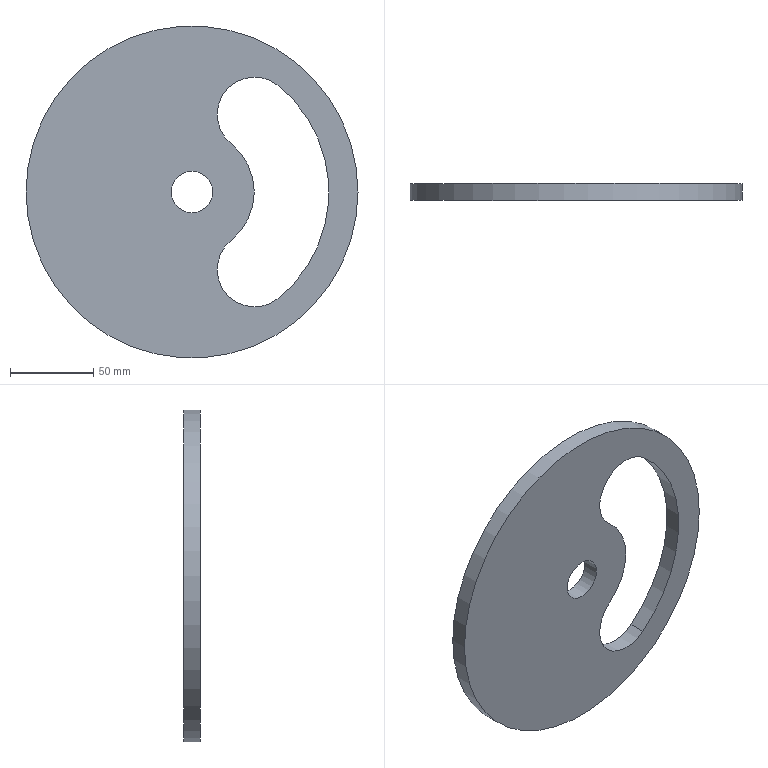Component | NX | VALVE_CORE | 1 solid | 8 faces | box 200 x 10 x 200 mm | volume 245200 mm3 | cylinder 6 | plane 2 | commonest cylinder face diameters 45 x2 75 x1 165 x1 200 x1 25 x1
STEP:
#1=CARTESIAN_POINT('',(0.,0.,0.));
#2=DIRECTION('',(0.,0.,1.));
#3=DIRECTION('',(1.,0.,0.));
#4=AXIS2_PLACEMENT_3D('',#1,#2,#3);
#5=CARTESIAN_POINT('',(51.825,-45.,-64.191));
#6=VERTEX_POINT('',#5);
#7=CARTESIAN_POINT('',(51.825,-35.,-64.191));
#8=VERTEX_POINT('',#7);
#9=CARTESIAN_POINT('',(51.825,-45.,-64.191));
#10=DIRECTION('',(0.,1.,0.));
#11=VECTOR('',#10,1.);
#12=LINE('',#9,#11);
#13=CARTESIAN_POINT('',(37.691,-45.,-46.684));
#14=DIRECTION('',(0.,1.,0.));
#15=DIRECTION('',(0.,0.,1.));
#16=AXIS2_PLACEMENT_3D('',#13,#14,#15);
#17=CYLINDRICAL_SURFACE('',#16,22.5);
#18=CARTESIAN_POINT('',(2.462,0.));
#19=DIRECTION('',(0.,1.));
#20=VECTOR('',#19,1.);
#21=LINE('',#18,#20);
#22=(GEOMETRIC_REPRESENTATION_CONTEXT(2)PARAMETRIC_REPRESENTATION_CONTEXT()REPRESENTATION_CONTEXT('',''));
#23=DEFINITIONAL_REPRESENTATION('',(#21),#22);
#24=PCURVE('',#17,#23);
#25=CARTESIAN_POINT('',(0.,-45.,0.));
#26=DIRECTION('',(0.,1.,0.));
#27=DIRECTION('',(0.,0.,1.));
#28=AXIS2_PLACEMENT_3D('',#25,#26,#27);
#29=CYLINDRICAL_SURFACE('',#28,82.5);
#30=CARTESIAN_POINT('',(2.462,0.));
#31=DIRECTION('',(0.,1.));
#32=VECTOR('',#31,1.);
#33=LINE('',#30,#32);
#34=(GEOMETRIC_REPRESENTATION_CONTEXT(2)PARAMETRIC_REPRESENTATION_CONTEXT()REPRESENTATION_CONTEXT('',''));
#35=DEFINITIONAL_REPRESENTATION('',(#33),#34);
#36=PCURVE('',#29,#35);
#37=SURFACE_CURVE('',#12,(#24,#36),.PCURVE_S1.);
#38=EDGE_CURVE('',#6,#8,#37,.T.);
#39=ORIENTED_EDGE('',*,*,#38,.F.);
#40=CARTESIAN_POINT('',(23.557,-45.,-29.178));
#41=VERTEX_POINT('',#40);
#42=CARTESIAN_POINT('',(37.691,-45.,-46.684));
#43=DIRECTION('',(0.,1.,0.));
#44=DIRECTION('',(1.,0.,0.));
#45=AXIS2_PLACEMENT_3D('',#42,#43,#44);
#46=CIRCLE('',#45,22.5);
#47=CARTESIAN_POINT('',(1.571,0.));
#48=DIRECTION('',(1.,0.));
#49=VECTOR('',#48,1.);
#50=LINE('',#47,#49);
#51=(GEOMETRIC_REPRESENTATION_CONTEXT(2)PARAMETRIC_REPRESENTATION_CONTEXT()REPRESENTATION_CONTEXT('',''));
#52=DEFINITIONAL_REPRESENTATION('',(#50),#51);
#53=PCURVE('',#17,#52);
#54=CARTESIAN_POINT('',(18.845,-45.,-23.342));
#55=DIRECTION('',(0.,-1.,0.));
#56=DIRECTION('',(0.,0.,-1.));
#57=AXIS2_PLACEMENT_3D('',#54,#55,#56);
#58=PLANE('',#57);
#59=CARTESIAN_POINT('',(23.342,41.345));
#60=CARTESIAN_POINT('',(62.313,41.345));
#61=CARTESIAN_POINT('',(42.828,7.595));
#62=CARTESIAN_POINT('',(23.342,-26.155));
#63=CARTESIAN_POINT('',(3.857,7.595));
#64=CARTESIAN_POINT('',(-15.629,41.345));
#65=CARTESIAN_POINT('',(23.342,41.345));
#66=(BOUNDED_CURVE()B_SPLINE_CURVE(2,(#59,#60,#61,#62,#63,#64,#65),.UNSPECIFIED.,.T.,.F.)B_SPLINE_CURVE_WITH_KNOTS((1,2,2,2,2,1),(-2.094,0.,2.094,4.189,6.283,8.378),.UNSPECIFIED.)CURVE()GEOMETRIC_REPRESENTATION_ITEM()RATIONAL_B_SPLINE_CURVE((1.,0.5,1.,0.5,1.,0.5,1.))REPRESENTATION_ITEM(''));
#67=(GEOMETRIC_REPRESENTATION_CONTEXT(2)PARAMETRIC_REPRESENTATION_CONTEXT()REPRESENTATION_CONTEXT('',''));
#68=DEFINITIONAL_REPRESENTATION('',(#66),#67);
#69=PCURVE('',#58,#68);
#70=SURFACE_CURVE('',#46,(#53,#69),.PCURVE_S1.);
#71=EDGE_CURVE('',#6,#41,#70,.T.);
#72=ORIENTED_EDGE('',*,*,#71,.T.);
#73=CARTESIAN_POINT('',(23.557,-35.,-29.178));
#74=VERTEX_POINT('',#73);
#75=CARTESIAN_POINT('',(23.557,-45.,-29.178));
#76=DIRECTION('',(0.,1.,0.));
#77=VECTOR('',#76,1.);
#78=LINE('',#75,#77);
#79=CARTESIAN_POINT('',(5.604,0.));
#80=DIRECTION('',(0.,1.));
#81=VECTOR('',#80,1.);
#82=LINE('',#79,#81);
#83=(GEOMETRIC_REPRESENTATION_CONTEXT(2)PARAMETRIC_REPRESENTATION_CONTEXT()REPRESENTATION_CONTEXT('',''));
#84=DEFINITIONAL_REPRESENTATION('',(#82),#83);
#85=PCURVE('',#17,#84);
#86=CARTESIAN_POINT('',(0.,-45.,0.));
#87=DIRECTION('',(0.,1.,0.));
#88=DIRECTION('',(0.,0.,1.));
#89=AXIS2_PLACEMENT_3D('',#86,#87,#88);
#90=CYLINDRICAL_SURFACE('',#89,37.5);
#91=CARTESIAN_POINT('',(2.462,0.));
#92=DIRECTION('',(0.,1.));
#93=VECTOR('',#92,1.);
#94=LINE('',#91,#93);
#95=(GEOMETRIC_REPRESENTATION_CONTEXT(2)PARAMETRIC_REPRESENTATION_CONTEXT()REPRESENTATION_CONTEXT('',''));
#96=DEFINITIONAL_REPRESENTATION('',(#94),#95);
#97=PCURVE('',#90,#96);
#98=SURFACE_CURVE('',#78,(#85,#97),.PCURVE_S1.);
#99=EDGE_CURVE('',#41,#74,#98,.T.);
#100=ORIENTED_EDGE('',*,*,#99,.T.);
#101=CARTESIAN_POINT('',(37.691,-35.,-46.684));
#102=DIRECTION('',(0.,1.,0.));
#103=DIRECTION('',(1.,0.,0.));
#104=AXIS2_PLACEMENT_3D('',#101,#102,#103);
#105=CIRCLE('',#104,22.5);
#106=CARTESIAN_POINT('',(1.571,10.));
#107=DIRECTION('',(1.,0.));
#108=VECTOR('',#107,1.);
#109=LINE('',#106,#108);
#110=(GEOMETRIC_REPRESENTATION_CONTEXT(2)PARAMETRIC_REPRESENTATION_CONTEXT()REPRESENTATION_CONTEXT('',''));
#111=DEFINITIONAL_REPRESENTATION('',(#109),#110);
#112=PCURVE('',#17,#111);
#113=CARTESIAN_POINT('',(18.845,-35.,-23.342));
#114=DIRECTION('',(0.,-1.,0.));
#115=DIRECTION('',(0.,0.,-1.));
#116=AXIS2_PLACEMENT_3D('',#113,#114,#115);
#117=PLANE('',#116);
#118=CARTESIAN_POINT('',(23.342,41.345));
#119=CARTESIAN_POINT('',(62.313,41.345));
#120=CARTESIAN_POINT('',(42.828,7.595));
#121=CARTESIAN_POINT('',(23.342,-26.155));
#122=CARTESIAN_POINT('',(3.857,7.595));
#123=CARTESIAN_POINT('',(-15.629,41.345));
#124=CARTESIAN_POINT('',(23.342,41.345));
#125=(BOUNDED_CURVE()B_SPLINE_CURVE(2,(#118,#119,#120,#121,#122,#123,#124),.UNSPECIFIED.,.T.,.F.)B_SPLINE_CURVE_WITH_KNOTS((1,2,2,2,2,1),(-2.094,0.,2.094,4.189,6.283,8.378),.UNSPECIFIED.)CURVE()GEOMETRIC_REPRESENTATION_ITEM()RATIONAL_B_SPLINE_CURVE((1.,0.5,1.,0.5,1.,0.5,1.))REPRESENTATION_ITEM(''));
#126=(GEOMETRIC_REPRESENTATION_CONTEXT(2)PARAMETRIC_REPRESENTATION_CONTEXT()REPRESENTATION_CONTEXT('',''));
#127=DEFINITIONAL_REPRESENTATION('',(#125),#126);
#128=PCURVE('',#117,#127);
#129=SURFACE_CURVE('',#105,(#112,#128),.PCURVE_S1.);
#130=EDGE_CURVE('',#8,#74,#129,.T.);
#131=ORIENTED_EDGE('',*,*,#130,.F.);
#132=EDGE_LOOP('',(#39,#72,#100,#131));
#133=FACE_BOUND('',#132,.F.);
#134=ADVANCED_FACE('',(#133),#17,.F.);
#135=CARTESIAN_POINT('',(23.557,-35.,29.178));
#136=VERTEX_POINT('',#135);
#137=CARTESIAN_POINT('',(0.,-35.,0.));
#138=DIRECTION('',(0.,-1.,0.));
#139=DIRECTION('',(1.,0.,-0.));
#140=AXIS2_PLACEMENT_3D('',#137,#138,#139);
#141=CIRCLE('',#140,37.5);
#142=CARTESIAN_POINT('',(7.854,10.));
#143=DIRECTION('',(-1.,0.));
#144=VECTOR('',#143,1.);
#145=LINE('',#142,#144);
#146=(GEOMETRIC_REPRESENTATION_CONTEXT(2)PARAMETRIC_REPRESENTATION_CONTEXT()REPRESENTATION_CONTEXT('',''));
#147=DEFINITIONAL_REPRESENTATION('',(#145),#146);
#148=PCURVE('',#90,#147);
#149=CARTESIAN_POINT('',(-23.342,-18.845));
#150=DIRECTION('',(0.,1.));
#151=AXIS2_PLACEMENT_2D('',#149,#150);
#152=CIRCLE('',#151,37.5);
#153=(GEOMETRIC_REPRESENTATION_CONTEXT(2)PARAMETRIC_REPRESENTATION_CONTEXT()REPRESENTATION_CONTEXT('',''));
#154=DEFINITIONAL_REPRESENTATION('',(#152),#153);
#155=PCURVE('',#117,#154);
#156=SURFACE_CURVE('',#141,(#148,#155),.PCURVE_S1.);
#157=EDGE_CURVE('',#74,#136,#156,.T.);
#158=ORIENTED_EDGE('',*,*,#157,.T.);
#159=CARTESIAN_POINT('',(23.557,-45.,29.178));
#160=VERTEX_POINT('',#159);
#161=CARTESIAN_POINT('',(23.557,-45.,29.178));
#162=DIRECTION('',(0.,1.,0.));
#163=VECTOR('',#162,1.);
#164=LINE('',#161,#163);
#165=CARTESIAN_POINT('',(0.6792,0.));
#166=DIRECTION('',(0.,1.));
#167=VECTOR('',#166,1.);
#168=LINE('',#165,#167);
#169=(GEOMETRIC_REPRESENTATION_CONTEXT(2)PARAMETRIC_REPRESENTATION_CONTEXT()REPRESENTATION_CONTEXT('',''));
#170=DEFINITIONAL_REPRESENTATION('',(#168),#169);
#171=PCURVE('',#90,#170);
#172=CARTESIAN_POINT('',(37.691,-45.,46.684));
#173=DIRECTION('',(0.,1.,0.));
#174=DIRECTION('',(0.,0.,1.));
#175=AXIS2_PLACEMENT_3D('',#172,#173,#174);
#176=CYLINDRICAL_SURFACE('',#175,22.5);
#177=CARTESIAN_POINT('',(3.821,0.));
#178=DIRECTION('',(0.,1.));
#179=VECTOR('',#178,1.);
#180=LINE('',#177,#179);
#181=(GEOMETRIC_REPRESENTATION_CONTEXT(2)PARAMETRIC_REPRESENTATION_CONTEXT()REPRESENTATION_CONTEXT('',''));
#182=DEFINITIONAL_REPRESENTATION('',(#180),#181);
#183=PCURVE('',#176,#182);
#184=SURFACE_CURVE('',#164,(#171,#183),.PCURVE_S1.);
#185=EDGE_CURVE('',#160,#136,#184,.T.);
#186=ORIENTED_EDGE('',*,*,#185,.F.);
#187=CARTESIAN_POINT('',(0.,-45.,0.));
#188=DIRECTION('',(0.,-1.,0.));
#189=DIRECTION('',(1.,0.,-0.));
#190=AXIS2_PLACEMENT_3D('',#187,#188,#189);
#191=CIRCLE('',#190,37.5);
#192=CARTESIAN_POINT('',(7.854,0.));
#193=DIRECTION('',(-1.,0.));
#194=VECTOR('',#193,1.);
#195=LINE('',#192,#194);
#196=(GEOMETRIC_REPRESENTATION_CONTEXT(2)PARAMETRIC_REPRESENTATION_CONTEXT()REPRESENTATION_CONTEXT('',''));
#197=DEFINITIONAL_REPRESENTATION('',(#195),#196);
#198=PCURVE('',#90,#197);
#199=CARTESIAN_POINT('',(-23.342,-18.845));
#200=DIRECTION('',(0.,1.));
#201=AXIS2_PLACEMENT_2D('',#199,#200);
#202=CIRCLE('',#201,37.5);
#203=(GEOMETRIC_REPRESENTATION_CONTEXT(2)PARAMETRIC_REPRESENTATION_CONTEXT()REPRESENTATION_CONTEXT('',''));
#204=DEFINITIONAL_REPRESENTATION('',(#202),#203);
#205=PCURVE('',#58,#204);
#206=SURFACE_CURVE('',#191,(#198,#205),.PCURVE_S1.);
#207=EDGE_CURVE('',#41,#160,#206,.T.);
#208=ORIENTED_EDGE('',*,*,#207,.F.);
#209=ORIENTED_EDGE('',*,*,#99,.T.);
#210=EDGE_LOOP('',(#158,#186,#208,#209));
#211=FACE_BOUND('',#210,.T.);
#212=ADVANCED_FACE('',(#211),#90,.T.);
#213=ORIENTED_EDGE('',*,*,#185,.F.);
#214=CARTESIAN_POINT('',(51.825,-45.,64.191));
#215=VERTEX_POINT('',#214);
#216=CARTESIAN_POINT('',(37.691,-45.,46.684));
#217=DIRECTION('',(0.,1.,0.));
#218=DIRECTION('',(0.7193,0.,-0.6947));
#219=AXIS2_PLACEMENT_3D('',#216,#217,#218);
#220=CIRCLE('',#219,22.5);
#221=CARTESIAN_POINT('',(2.339,0.));
#222=DIRECTION('',(1.,0.));
#223=VECTOR('',#222,1.);
#224=LINE('',#221,#223);
#225=(GEOMETRIC_REPRESENTATION_CONTEXT(2)PARAMETRIC_REPRESENTATION_CONTEXT()REPRESENTATION_CONTEXT('',''));
#226=DEFINITIONAL_REPRESENTATION('',(#224),#225);
#227=PCURVE('',#176,#226);
#228=CARTESIAN_POINT('',(-54.397,35.03));
#229=CARTESIAN_POINT('',(-26.363,7.959));
#230=CARTESIAN_POINT('',(-63.825,-2.783));
#231=CARTESIAN_POINT('',(-101.286,-13.525));
#232=CARTESIAN_POINT('',(-91.858,24.289));
#233=CARTESIAN_POINT('',(-82.43,62.102));
#234=CARTESIAN_POINT('',(-54.397,35.03));
#235=(BOUNDED_CURVE()B_SPLINE_CURVE(2,(#228,#229,#230,#231,#232,#233,#234),.UNSPECIFIED.,.T.,.F.)B_SPLINE_CURVE_WITH_KNOTS((1,2,2,2,2,1),(-2.094,0.,2.094,4.189,6.283,8.378),.UNSPECIFIED.)CURVE()GEOMETRIC_REPRESENTATION_ITEM()RATIONAL_B_SPLINE_CURVE((1.,0.5,1.,0.5,1.,0.5,1.))REPRESENTATION_ITEM(''));
#236=(GEOMETRIC_REPRESENTATION_CONTEXT(2)PARAMETRIC_REPRESENTATION_CONTEXT()REPRESENTATION_CONTEXT('',''));
#237=DEFINITIONAL_REPRESENTATION('',(#235),#236);
#238=PCURVE('',#58,#237);
#239=SURFACE_CURVE('',#220,(#227,#238),.PCURVE_S1.);
#240=EDGE_CURVE('',#160,#215,#239,.T.);
#241=ORIENTED_EDGE('',*,*,#240,.T.);
#242=CARTESIAN_POINT('',(51.825,-35.,64.191));
#243=VERTEX_POINT('',#242);
#244=CARTESIAN_POINT('',(51.825,-45.,64.191));
#245=DIRECTION('',(0.,1.,0.));
#246=VECTOR('',#245,1.);
#247=LINE('',#244,#246);
#248=CARTESIAN_POINT('',(6.962,0.));
#249=DIRECTION('',(0.,1.));
#250=VECTOR('',#249,1.);
#251=LINE('',#248,#250);
#252=(GEOMETRIC_REPRESENTATION_CONTEXT(2)PARAMETRIC_REPRESENTATION_CONTEXT()REPRESENTATION_CONTEXT('',''));
#253=DEFINITIONAL_REPRESENTATION('',(#251),#252);
#254=PCURVE('',#176,#253);
#255=CARTESIAN_POINT('',(0.6792,0.));
#256=DIRECTION('',(0.,1.));
#257=VECTOR('',#256,1.);
#258=LINE('',#255,#257);
#259=(GEOMETRIC_REPRESENTATION_CONTEXT(2)PARAMETRIC_REPRESENTATION_CONTEXT()REPRESENTATION_CONTEXT('',''));
#260=DEFINITIONAL_REPRESENTATION('',(#258),#259);
#261=PCURVE('',#29,#260);
#262=SURFACE_CURVE('',#247,(#254,#261),.PCURVE_S1.);
#263=EDGE_CURVE('',#215,#243,#262,.T.);
#264=ORIENTED_EDGE('',*,*,#263,.T.);
#265=CARTESIAN_POINT('',(37.691,-35.,46.684));
#266=DIRECTION('',(0.,1.,0.));
#267=DIRECTION('',(0.7193,0.,-0.6947));
#268=AXIS2_PLACEMENT_3D('',#265,#266,#267);
#269=CIRCLE('',#268,22.5);
#270=CARTESIAN_POINT('',(2.339,10.));
#271=DIRECTION('',(1.,0.));
#272=VECTOR('',#271,1.);
#273=LINE('',#270,#272);
#274=(GEOMETRIC_REPRESENTATION_CONTEXT(2)PARAMETRIC_REPRESENTATION_CONTEXT()REPRESENTATION_CONTEXT('',''));
#275=DEFINITIONAL_REPRESENTATION('',(#273),#274);
#276=PCURVE('',#176,#275);
#277=CARTESIAN_POINT('',(-54.397,35.03));
#278=CARTESIAN_POINT('',(-26.363,7.959));
#279=CARTESIAN_POINT('',(-63.825,-2.783));
#280=CARTESIAN_POINT('',(-101.286,-13.525));
#281=CARTESIAN_POINT('',(-91.858,24.289));
#282=CARTESIAN_POINT('',(-82.43,62.102));
#283=CARTESIAN_POINT('',(-54.397,35.03));
#284=(BOUNDED_CURVE()B_SPLINE_CURVE(2,(#277,#278,#279,#280,#281,#282,#283),.UNSPECIFIED.,.T.,.F.)B_SPLINE_CURVE_WITH_KNOTS((1,2,2,2,2,1),(-2.094,0.,2.094,4.189,6.283,8.378),.UNSPECIFIED.)CURVE()GEOMETRIC_REPRESENTATION_ITEM()RATIONAL_B_SPLINE_CURVE((1.,0.5,1.,0.5,1.,0.5,1.))REPRESENTATION_ITEM(''));
#285=(GEOMETRIC_REPRESENTATION_CONTEXT(2)PARAMETRIC_REPRESENTATION_CONTEXT()REPRESENTATION_CONTEXT('',''));
#286=DEFINITIONAL_REPRESENTATION('',(#284),#285);
#287=PCURVE('',#117,#286);
#288=SURFACE_CURVE('',#269,(#276,#287),.PCURVE_S1.);
#289=EDGE_CURVE('',#136,#243,#288,.T.);
#290=ORIENTED_EDGE('',*,*,#289,.F.);
#291=EDGE_LOOP('',(#213,#241,#264,#290));
#292=FACE_BOUND('',#291,.F.);
#293=ADVANCED_FACE('',(#292),#176,.F.);
#294=ORIENTED_EDGE('',*,*,#263,.F.);
#295=CARTESIAN_POINT('',(0.,-45.,0.));
#296=DIRECTION('',(0.,1.,0.));
#297=DIRECTION('',(1.,0.,0.));
#298=AXIS2_PLACEMENT_3D('',#295,#296,#297);
#299=CIRCLE('',#298,82.5);
#300=CARTESIAN_POINT('',(-4.712,0.));
#301=DIRECTION('',(1.,0.));
#302=VECTOR('',#301,1.);
#303=LINE('',#300,#302);
#304=(GEOMETRIC_REPRESENTATION_CONTEXT(2)PARAMETRIC_REPRESENTATION_CONTEXT()REPRESENTATION_CONTEXT('',''));
#305=DEFINITIONAL_REPRESENTATION('',(#303),#304);
#306=PCURVE('',#29,#305);
#307=CARTESIAN_POINT('',(-23.342,63.655));
#308=CARTESIAN_POINT('',(119.552,63.655));
#309=CARTESIAN_POINT('',(48.105,-60.095));
#310=CARTESIAN_POINT('',(-23.342,-183.845));
#311=CARTESIAN_POINT('',(-94.789,-60.095));
#312=CARTESIAN_POINT('',(-166.236,63.655));
#313=CARTESIAN_POINT('',(-23.342,63.655));
#314=(BOUNDED_CURVE()B_SPLINE_CURVE(2,(#307,#308,#309,#310,#311,#312,#313),.UNSPECIFIED.,.T.,.F.)B_SPLINE_CURVE_WITH_KNOTS((1,2,2,2,2,1),(-2.094,0.,2.094,4.189,6.283,8.378),.UNSPECIFIED.)CURVE()GEOMETRIC_REPRESENTATION_ITEM()RATIONAL_B_SPLINE_CURVE((1.,0.5,1.,0.5,1.,0.5,1.))REPRESENTATION_ITEM(''));
#315=(GEOMETRIC_REPRESENTATION_CONTEXT(2)PARAMETRIC_REPRESENTATION_CONTEXT()REPRESENTATION_CONTEXT('',''));
#316=DEFINITIONAL_REPRESENTATION('',(#314),#315);
#317=PCURVE('',#58,#316);
#318=SURFACE_CURVE('',#299,(#306,#317),.PCURVE_S1.);
#319=EDGE_CURVE('',#215,#6,#318,.T.);
#320=ORIENTED_EDGE('',*,*,#319,.T.);
#321=ORIENTED_EDGE('',*,*,#38,.T.);
#322=CARTESIAN_POINT('',(0.,-35.,0.));
#323=DIRECTION('',(0.,1.,0.));
#324=DIRECTION('',(1.,0.,0.));
#325=AXIS2_PLACEMENT_3D('',#322,#323,#324);
#326=CIRCLE('',#325,82.5);
#327=CARTESIAN_POINT('',(-4.712,10.));
#328=DIRECTION('',(1.,0.));
#329=VECTOR('',#328,1.);
#330=LINE('',#327,#329);
#331=(GEOMETRIC_REPRESENTATION_CONTEXT(2)PARAMETRIC_REPRESENTATION_CONTEXT()REPRESENTATION_CONTEXT('',''));
#332=DEFINITIONAL_REPRESENTATION('',(#330),#331);
#333=PCURVE('',#29,#332);
#334=CARTESIAN_POINT('',(-23.342,63.655));
#335=CARTESIAN_POINT('',(119.552,63.655));
#336=CARTESIAN_POINT('',(48.105,-60.095));
#337=CARTESIAN_POINT('',(-23.342,-183.845));
#338=CARTESIAN_POINT('',(-94.789,-60.095));
#339=CARTESIAN_POINT('',(-166.236,63.655));
#340=CARTESIAN_POINT('',(-23.342,63.655));
#341=(BOUNDED_CURVE()B_SPLINE_CURVE(2,(#334,#335,#336,#337,#338,#339,#340),.UNSPECIFIED.,.T.,.F.)B_SPLINE_CURVE_WITH_KNOTS((1,2,2,2,2,1),(-2.094,0.,2.094,4.189,6.283,8.378),.UNSPECIFIED.)CURVE()GEOMETRIC_REPRESENTATION_ITEM()RATIONAL_B_SPLINE_CURVE((1.,0.5,1.,0.5,1.,0.5,1.))REPRESENTATION_ITEM(''));
#342=(GEOMETRIC_REPRESENTATION_CONTEXT(2)PARAMETRIC_REPRESENTATION_CONTEXT()REPRESENTATION_CONTEXT('',''));
#343=DEFINITIONAL_REPRESENTATION('',(#341),#342);
#344=PCURVE('',#117,#343);
#345=SURFACE_CURVE('',#326,(#333,#344),.PCURVE_S1.);
#346=EDGE_CURVE('',#243,#8,#345,.T.);
#347=ORIENTED_EDGE('',*,*,#346,.F.);
#348=EDGE_LOOP('',(#294,#320,#321,#347));
#349=FACE_BOUND('',#348,.F.);
#350=ADVANCED_FACE('',(#349),#29,.F.);
#351=CARTESIAN_POINT('',(100.,-45.,-0.));
#352=VERTEX_POINT('',#351);
#353=CARTESIAN_POINT('',(0.,-45.,0.));
#354=DIRECTION('',(0.,-1.,0.));
#355=DIRECTION('',(1.,0.,-0.));
#356=AXIS2_PLACEMENT_3D('',#353,#354,#355);
#357=CIRCLE('',#356,100.);
#358=CARTESIAN_POINT('',(0.,-45.,0.));
#359=DIRECTION('',(0.,1.,0.));
#360=DIRECTION('',(0.,0.,1.));
#361=AXIS2_PLACEMENT_3D('',#358,#359,#360);
#362=CYLINDRICAL_SURFACE('',#361,100.);
#363=CARTESIAN_POINT('',(7.854,0.));
#364=DIRECTION('',(-1.,0.));
#365=VECTOR('',#364,1.);
#366=LINE('',#363,#365);
#367=(GEOMETRIC_REPRESENTATION_CONTEXT(2)PARAMETRIC_REPRESENTATION_CONTEXT()REPRESENTATION_CONTEXT('',''));
#368=DEFINITIONAL_REPRESENTATION('',(#366),#367);
#369=PCURVE('',#362,#368);
#370=CARTESIAN_POINT('',(-23.342,-18.845));
#371=DIRECTION('',(0.,1.));
#372=AXIS2_PLACEMENT_2D('',#370,#371);
#373=CIRCLE('',#372,100.);
#374=(GEOMETRIC_REPRESENTATION_CONTEXT(2)PARAMETRIC_REPRESENTATION_CONTEXT()REPRESENTATION_CONTEXT('',''));
#375=DEFINITIONAL_REPRESENTATION('',(#373),#374);
#376=PCURVE('',#58,#375);
#377=SURFACE_CURVE('',#357,(#369,#376),.PCURVE_S1.);
#378=EDGE_CURVE('',#352,#352,#377,.T.);
#379=ORIENTED_EDGE('',*,*,#378,.F.);
#380=CARTESIAN_POINT('',(100.,-35.,-0.));
#381=VERTEX_POINT('',#380);
#382=CARTESIAN_POINT('',(100.,-45.,0.));
#383=CARTESIAN_POINT('',(100.,-35.,0.));
#384=B_SPLINE_CURVE_WITH_KNOTS('',1,(#382,#383),.UNSPECIFIED.,.F.,.F.,(2,2),(0.,10.),.PIECEWISE_BEZIER_KNOTS.);
#385=CARTESIAN_POINT('',(7.854,0.));
#386=DIRECTION('',(0.,1.));
#387=VECTOR('',#386,1.);
#388=LINE('',#385,#387);
#389=(GEOMETRIC_REPRESENTATION_CONTEXT(2)PARAMETRIC_REPRESENTATION_CONTEXT()REPRESENTATION_CONTEXT('',''));
#390=DEFINITIONAL_REPRESENTATION('',(#388),#389);
#391=PCURVE('',#362,#390);
#392=CARTESIAN_POINT('',(1.571,0.));
#393=DIRECTION('',(0.,1.));
#394=VECTOR('',#393,1.);
#395=LINE('',#392,#394);
#396=(GEOMETRIC_REPRESENTATION_CONTEXT(2)PARAMETRIC_REPRESENTATION_CONTEXT()REPRESENTATION_CONTEXT('',''));
#397=DEFINITIONAL_REPRESENTATION('',(#395),#396);
#398=PCURVE('',#362,#397);
#399=SEAM_CURVE('',#384,(#391,#398),.PCURVE_S1.);
#400=EDGE_CURVE('',#352,#381,#399,.T.);
#401=ORIENTED_EDGE('',*,*,#400,.T.);
#402=CARTESIAN_POINT('',(0.,-35.,0.));
#403=DIRECTION('',(0.,-1.,0.));
#404=DIRECTION('',(1.,0.,-0.));
#405=AXIS2_PLACEMENT_3D('',#402,#403,#404);
#406=CIRCLE('',#405,100.);
#407=CARTESIAN_POINT('',(7.854,10.));
#408=DIRECTION('',(-1.,0.));
#409=VECTOR('',#408,1.);
#410=LINE('',#407,#409);
#411=(GEOMETRIC_REPRESENTATION_CONTEXT(2)PARAMETRIC_REPRESENTATION_CONTEXT()REPRESENTATION_CONTEXT('',''));
#412=DEFINITIONAL_REPRESENTATION('',(#410),#411);
#413=PCURVE('',#362,#412);
#414=CARTESIAN_POINT('',(-23.342,-18.845));
#415=DIRECTION('',(0.,1.));
#416=AXIS2_PLACEMENT_2D('',#414,#415);
#417=CIRCLE('',#416,100.);
#418=(GEOMETRIC_REPRESENTATION_CONTEXT(2)PARAMETRIC_REPRESENTATION_CONTEXT()REPRESENTATION_CONTEXT('',''));
#419=DEFINITIONAL_REPRESENTATION('',(#417),#418);
#420=PCURVE('',#117,#419);
#421=SURFACE_CURVE('',#406,(#413,#420),.PCURVE_S1.);
#422=EDGE_CURVE('',#381,#381,#421,.T.);
#423=ORIENTED_EDGE('',*,*,#422,.T.);
#424=ORIENTED_EDGE('',*,*,#400,.F.);
#425=EDGE_LOOP('',(#379,#401,#423,#424));
#426=FACE_BOUND('',#425,.T.);
#427=ADVANCED_FACE('',(#426),#362,.T.);
#428=CARTESIAN_POINT('',(0.,-45.,-12.5));
#429=VERTEX_POINT('',#428);
#430=CARTESIAN_POINT('',(0.,-45.,0.));
#431=DIRECTION('',(0.,1.,0.));
#432=DIRECTION('',(0.,0.,-1.));
#433=AXIS2_PLACEMENT_3D('',#430,#431,#432);
#434=CIRCLE('',#433,12.5);
#435=CARTESIAN_POINT('',(0.,87.,0.));
#436=DIRECTION('',(0.,-1.,0.));
#437=DIRECTION('',(0.,0.,-1.));
#438=AXIS2_PLACEMENT_3D('',#435,#436,#437);
#439=CYLINDRICAL_SURFACE('',#438,12.5);
#440=CARTESIAN_POINT('',(6.283,132.));
#441=DIRECTION('',(-1.,0.));
#442=VECTOR('',#441,1.);
#443=LINE('',#440,#442);
#444=(GEOMETRIC_REPRESENTATION_CONTEXT(2)PARAMETRIC_REPRESENTATION_CONTEXT()REPRESENTATION_CONTEXT('',''));
#445=DEFINITIONAL_REPRESENTATION('',(#443),#444);
#446=PCURVE('',#439,#445);
#447=CARTESIAN_POINT('',(-10.842,-18.845));
#448=CARTESIAN_POINT('',(-10.842,-40.496));
#449=CARTESIAN_POINT('',(-29.592,-29.671));
#450=CARTESIAN_POINT('',(-48.342,-18.845));
#451=CARTESIAN_POINT('',(-29.592,-8.02));
#452=CARTESIAN_POINT('',(-10.842,2.805));
#453=CARTESIAN_POINT('',(-10.842,-18.845));
#454=(BOUNDED_CURVE()B_SPLINE_CURVE(2,(#447,#448,#449,#450,#451,#452,#453),.UNSPECIFIED.,.T.,.F.)B_SPLINE_CURVE_WITH_KNOTS((1,2,2,2,2,1),(-2.094,0.,2.094,4.189,6.283,8.378),.UNSPECIFIED.)CURVE()GEOMETRIC_REPRESENTATION_ITEM()RATIONAL_B_SPLINE_CURVE((1.,0.5,1.,0.5,1.,0.5,1.))REPRESENTATION_ITEM(''));
#455=(GEOMETRIC_REPRESENTATION_CONTEXT(2)PARAMETRIC_REPRESENTATION_CONTEXT()REPRESENTATION_CONTEXT('',''));
#456=DEFINITIONAL_REPRESENTATION('',(#454),#455);
#457=PCURVE('',#58,#456);
#458=SURFACE_CURVE('',#434,(#446,#457),.PCURVE_S1.);
#459=EDGE_CURVE('',#429,#429,#458,.T.);
#460=ORIENTED_EDGE('',*,*,#459,.T.);
#461=CARTESIAN_POINT('',(0.,-35.,-12.5));
#462=VERTEX_POINT('',#461);
#463=CARTESIAN_POINT('',(-0.,-35.,-12.5));
#464=CARTESIAN_POINT('',(-0.,-45.,-12.5));
#465=B_SPLINE_CURVE_WITH_KNOTS('',1,(#463,#464),.UNSPECIFIED.,.F.,.F.,(2,2),(122.,132.),.PIECEWISE_BEZIER_KNOTS.);
#466=CARTESIAN_POINT('',(0.,0.));
#467=DIRECTION('',(0.,1.));
#468=VECTOR('',#467,1.);
#469=LINE('',#466,#468);
#470=(GEOMETRIC_REPRESENTATION_CONTEXT(2)PARAMETRIC_REPRESENTATION_CONTEXT()REPRESENTATION_CONTEXT('',''));
#471=DEFINITIONAL_REPRESENTATION('',(#469),#470);
#472=PCURVE('',#439,#471);
#473=CARTESIAN_POINT('',(6.283,0.));
#474=DIRECTION('',(0.,1.));
#475=VECTOR('',#474,1.);
#476=LINE('',#473,#475);
#477=(GEOMETRIC_REPRESENTATION_CONTEXT(2)PARAMETRIC_REPRESENTATION_CONTEXT()REPRESENTATION_CONTEXT('',''));
#478=DEFINITIONAL_REPRESENTATION('',(#476),#477);
#479=PCURVE('',#439,#478);
#480=SEAM_CURVE('',#465,(#472,#479),.PCURVE_S1.);
#481=EDGE_CURVE('',#462,#429,#480,.T.);
#482=ORIENTED_EDGE('',*,*,#481,.F.);
#483=CARTESIAN_POINT('',(0.,-35.,0.));
#484=DIRECTION('',(0.,1.,0.));
#485=DIRECTION('',(0.,0.,-1.));
#486=AXIS2_PLACEMENT_3D('',#483,#484,#485);
#487=CIRCLE('',#486,12.5);
#488=CARTESIAN_POINT('',(6.283,122.));
#489=DIRECTION('',(-1.,0.));
#490=VECTOR('',#489,1.);
#491=LINE('',#488,#490);
#492=(GEOMETRIC_REPRESENTATION_CONTEXT(2)PARAMETRIC_REPRESENTATION_CONTEXT()REPRESENTATION_CONTEXT('',''));
#493=DEFINITIONAL_REPRESENTATION('',(#491),#492);
#494=PCURVE('',#439,#493);
#495=CARTESIAN_POINT('',(-10.842,-18.845));
#496=CARTESIAN_POINT('',(-10.842,-40.496));
#497=CARTESIAN_POINT('',(-29.592,-29.671));
#498=CARTESIAN_POINT('',(-48.342,-18.845));
#499=CARTESIAN_POINT('',(-29.592,-8.02));
#500=CARTESIAN_POINT('',(-10.842,2.805));
#501=CARTESIAN_POINT('',(-10.842,-18.845));
#502=(BOUNDED_CURVE()B_SPLINE_CURVE(2,(#495,#496,#497,#498,#499,#500,#501),.UNSPECIFIED.,.T.,.F.)B_SPLINE_CURVE_WITH_KNOTS((1,2,2,2,2,1),(-2.094,0.,2.094,4.189,6.283,8.378),.UNSPECIFIED.)CURVE()GEOMETRIC_REPRESENTATION_ITEM()RATIONAL_B_SPLINE_CURVE((1.,0.5,1.,0.5,1.,0.5,1.))REPRESENTATION_ITEM(''));
#503=(GEOMETRIC_REPRESENTATION_CONTEXT(2)PARAMETRIC_REPRESENTATION_CONTEXT()REPRESENTATION_CONTEXT('',''));
#504=DEFINITIONAL_REPRESENTATION('',(#502),#503);
#505=PCURVE('',#117,#504);
#506=SURFACE_CURVE('',#487,(#494,#505),.PCURVE_S1.);
#507=EDGE_CURVE('',#462,#462,#506,.T.);
#508=ORIENTED_EDGE('',*,*,#507,.F.);
#509=ORIENTED_EDGE('',*,*,#481,.T.);
#510=EDGE_LOOP('',(#460,#482,#508,#509));
#511=FACE_BOUND('',#510,.F.);
#512=ADVANCED_FACE('',(#511),#439,.F.);
#513=ORIENTED_EDGE('',*,*,#378,.T.);
#514=EDGE_LOOP('',(#513));
#515=FACE_BOUND('',#514,.T.);
#516=ORIENTED_EDGE('',*,*,#71,.T.);
#517=ORIENTED_EDGE('',*,*,#207,.T.);
#518=ORIENTED_EDGE('',*,*,#240,.T.);
#519=ORIENTED_EDGE('',*,*,#319,.T.);
#520=EDGE_LOOP('',(#516,#517,#518,#519));
#521=FACE_BOUND('',#520,.T.);
#522=ORIENTED_EDGE('',*,*,#459,.T.);
#523=EDGE_LOOP('',(#522));
#524=FACE_BOUND('',#523,.T.);
#525=ADVANCED_FACE('',(#515,#521,#524),#58,.T.);
#526=ORIENTED_EDGE('',*,*,#422,.F.);
#527=EDGE_LOOP('',(#526));
#528=FACE_BOUND('',#527,.T.);
#529=ORIENTED_EDGE('',*,*,#130,.F.);
#530=ORIENTED_EDGE('',*,*,#346,.F.);
#531=ORIENTED_EDGE('',*,*,#289,.F.);
#532=ORIENTED_EDGE('',*,*,#157,.F.);
#533=EDGE_LOOP('',(#529,#530,#531,#532));
#534=FACE_BOUND('',#533,.T.);
#535=ORIENTED_EDGE('',*,*,#507,.F.);
#536=EDGE_LOOP('',(#535));
#537=FACE_BOUND('',#536,.T.);
#538=ADVANCED_FACE('',(#528,#534,#537),#117,.F.);
#539=CLOSED_SHELL('',(#134,#212,#293,#350,#427,#512,#525,#538));
#540=MANIFOLD_SOLID_BREP('',#539);
#541=(LENGTH_UNIT()NAMED_UNIT(*)SI_UNIT(.MILLI.,.METRE.));
#542=UNCERTAINTY_MEASURE_WITH_UNIT(LENGTH_MEASURE(0.000002),#541,'','');
#543=(NAMED_UNIT(*)PLANE_ANGLE_UNIT()SI_UNIT($,.RADIAN.));
#544=(NAMED_UNIT(*)SI_UNIT($,.STERADIAN.)SOLID_ANGLE_UNIT());
#545=(GEOMETRIC_REPRESENTATION_CONTEXT(3)GLOBAL_UNCERTAINTY_ASSIGNED_CONTEXT((#542))GLOBAL_UNIT_ASSIGNED_CONTEXT((#541,#543,#544))REPRESENTATION_CONTEXT('',''));
#546=ADVANCED_BREP_SHAPE_REPRESENTATION('',(#4,#540),#545);